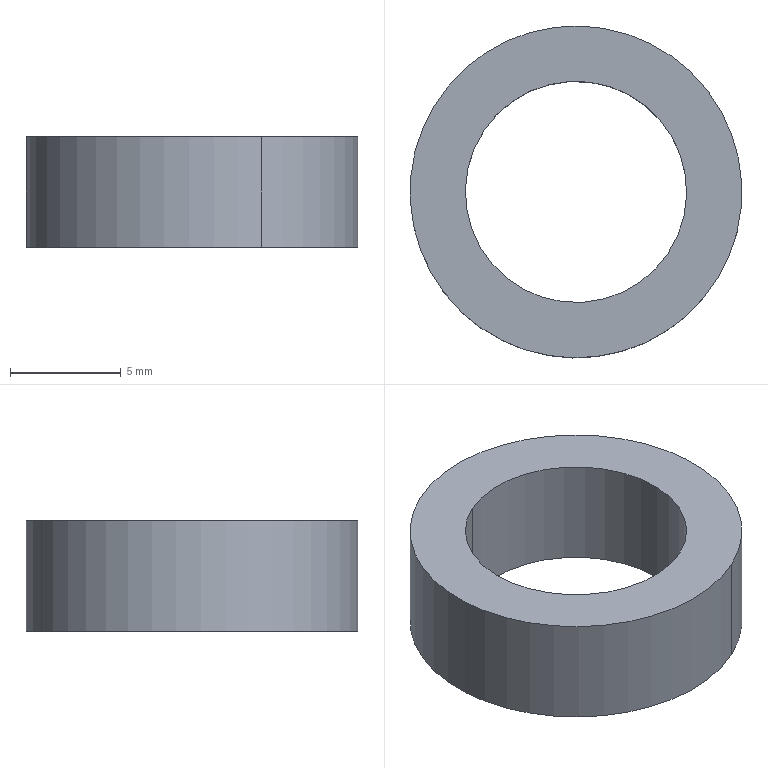Component | SolidWorks | RetainingRing-3 | 1 solid | 6 faces | box 15 x 15 x 5 mm | volume 491 mm3 | cylinder 4 | plane 2 | commonest cylinder face diameters 10 x2 15 x2
build123d program:
from build123d import *

# Parameters (mm, degrees)
SKETCH1_R           = 7.5
SKETCH1_R_2         = 5
BOSS_EXTRUDE1_DEPTH = 5


with BuildPart() as part:
    # Sketch1 → Boss-Extrude1 (new body)
    with BuildSketch(Plane.XY):
        with Locations((215.746, 95.507)):
            Circle(SKETCH1_R)
        with Locations((215.746, 95.507)):
            Circle(SKETCH1_R_2, mode=Mode.SUBTRACT)
    extrude(amount=BOSS_EXTRUDE1_DEPTH)


solid = part.part

# Placed as in the assembly
solid = solid.moved(Location((-435.956, -47.976, -42.818), (0, 0, 0)))
STEP:
#1=COLOUR_RGB('',0.7922,0.8196,0.9333);
#2=FILL_AREA_STYLE_COLOUR('',#1);
#3=FILL_AREA_STYLE('',(#2));
#4=SURFACE_STYLE_FILL_AREA(#3);
#5=SURFACE_SIDE_STYLE('',(#4));
#6=SURFACE_STYLE_USAGE(.BOTH.,#5);
#7=PRESENTATION_STYLE_ASSIGNMENT((#6));
#8=CARTESIAN_POINT('',(-8.752,2.05,-1.686));
#9=VERTEX_POINT('',#8);
#10=CARTESIAN_POINT('',(-8.588,1.692,-1.686));
#11=VERTEX_POINT('',#10);
#12=CARTESIAN_POINT('',(-8.67,1.871,-1.686));
#13=DIRECTION('',(0.,-0.,-1.));
#14=DIRECTION('',(0.4168,-0.909,0.));
#15=AXIS2_PLACEMENT_3D('',#12,#13,#14);
#16=CIRCLE('',#15,0.1969);
#17=EDGE_CURVE('',#9,#11,#16,.T.);
#18=ORIENTED_EDGE('',*,*,#17,.T.);
#19=CARTESIAN_POINT('',(-8.588,1.692,-1.489));
#20=VERTEX_POINT('',#19);
#21=CARTESIAN_POINT('',(-8.588,1.692,-1.686));
#22=DIRECTION('',(-0.,0.,1.));
#23=VECTOR('',#22,39.37);
#24=LINE('',#21,#23);
#25=EDGE_CURVE('',#11,#20,#24,.T.);
#26=ORIENTED_EDGE('',*,*,#25,.T.);
#27=CARTESIAN_POINT('',(-8.752,2.05,-1.489));
#28=VERTEX_POINT('',#27);
#29=CARTESIAN_POINT('',(-8.67,1.871,-1.489));
#30=DIRECTION('',(0.,-0.,-1.));
#31=DIRECTION('',(0.4168,-0.909,0.));
#32=AXIS2_PLACEMENT_3D('',#29,#30,#31);
#33=CIRCLE('',#32,0.1969);
#34=EDGE_CURVE('',#28,#20,#33,.T.);
#35=ORIENTED_EDGE('',*,*,#34,.F.);
#36=CARTESIAN_POINT('',(-8.752,2.05,-1.686));
#37=DIRECTION('',(-0.,0.,1.));
#38=VECTOR('',#37,39.37);
#39=LINE('',#36,#38);
#40=EDGE_CURVE('',#9,#28,#39,.T.);
#41=ORIENTED_EDGE('',*,*,#40,.F.);
#42=EDGE_LOOP('',(#18,#26,#35,#41));
#43=FACE_OUTER_BOUND('',#42,.T.);
#44=CARTESIAN_POINT('',(-8.67,1.871,-1.686));
#45=DIRECTION('',(-0.,0.,1.));
#46=DIRECTION('',(-0.4168,0.909,0.));
#47=AXIS2_PLACEMENT_3D('',#44,#45,#46);
#48=CYLINDRICAL_SURFACE('',#47,0.1969);
#49=ADVANCED_FACE('',(#43),#48,.F.);
#50=CARTESIAN_POINT('',(-8.547,1.603,-1.686));
#51=VERTEX_POINT('',#50);
#52=CARTESIAN_POINT('',(-8.793,2.14,-1.686));
#53=VERTEX_POINT('',#52);
#54=CARTESIAN_POINT('',(-8.67,1.871,-1.686));
#55=DIRECTION('',(0.,-0.,-1.));
#56=DIRECTION('',(0.4168,-0.909,0.));
#57=AXIS2_PLACEMENT_3D('',#54,#55,#56);
#58=CIRCLE('',#57,0.2953);
#59=EDGE_CURVE('',#51,#53,#58,.T.);
#60=ORIENTED_EDGE('',*,*,#59,.F.);
#61=CARTESIAN_POINT('',(-8.547,1.603,-1.489));
#62=VERTEX_POINT('',#61);
#63=CARTESIAN_POINT('',(-8.547,1.603,-1.686));
#64=DIRECTION('',(-0.,0.,1.));
#65=VECTOR('',#64,39.37);
#66=LINE('',#63,#65);
#67=EDGE_CURVE('',#51,#62,#66,.T.);
#68=ORIENTED_EDGE('',*,*,#67,.T.);
#69=CARTESIAN_POINT('',(-8.793,2.14,-1.489));
#70=VERTEX_POINT('',#69);
#71=CARTESIAN_POINT('',(-8.67,1.871,-1.489));
#72=DIRECTION('',(0.,-0.,-1.));
#73=DIRECTION('',(0.4168,-0.909,0.));
#74=AXIS2_PLACEMENT_3D('',#71,#72,#73);
#75=CIRCLE('',#74,0.2953);
#76=EDGE_CURVE('',#62,#70,#75,.T.);
#77=ORIENTED_EDGE('',*,*,#76,.T.);
#78=CARTESIAN_POINT('',(-8.793,2.14,-1.686));
#79=DIRECTION('',(-0.,0.,1.));
#80=VECTOR('',#79,39.37);
#81=LINE('',#78,#80);
#82=EDGE_CURVE('',#53,#70,#81,.T.);
#83=ORIENTED_EDGE('',*,*,#82,.F.);
#84=EDGE_LOOP('',(#60,#68,#77,#83));
#85=FACE_OUTER_BOUND('',#84,.T.);
#86=CARTESIAN_POINT('',(-8.67,1.871,-1.686));
#87=DIRECTION('',(-0.,0.,1.));
#88=DIRECTION('',(-0.4168,0.909,0.));
#89=AXIS2_PLACEMENT_3D('',#86,#87,#88);
#90=CYLINDRICAL_SURFACE('',#89,0.2953);
#91=ADVANCED_FACE('',(#85),#90,.T.);
#92=CARTESIAN_POINT('',(-8.67,1.871,-1.686));
#93=DIRECTION('',(0.,-0.,-1.));
#94=DIRECTION('',(0.4168,-0.909,0.));
#95=AXIS2_PLACEMENT_3D('',#92,#93,#94);
#96=CIRCLE('',#95,0.2953);
#97=EDGE_CURVE('',#53,#51,#96,.T.);
#98=ORIENTED_EDGE('',*,*,#97,.T.);
#99=ORIENTED_EDGE('',*,*,#59,.T.);
#100=EDGE_LOOP('',(#98,#99));
#101=FACE_OUTER_BOUND('',#100,.T.);
#102=ORIENTED_EDGE('',*,*,#17,.F.);
#103=CARTESIAN_POINT('',(-8.67,1.871,-1.686));
#104=DIRECTION('',(0.,-0.,-1.));
#105=DIRECTION('',(0.4168,-0.909,0.));
#106=AXIS2_PLACEMENT_3D('',#103,#104,#105);
#107=CIRCLE('',#106,0.1969);
#108=EDGE_CURVE('',#11,#9,#107,.T.);
#109=ORIENTED_EDGE('',*,*,#108,.F.);
#110=EDGE_LOOP('',(#102,#109));
#111=FACE_BOUND('',#110,.T.);
#112=CARTESIAN_POINT('',(-8.67,1.871,-1.686));
#113=DIRECTION('',(0.,-0.,-1.));
#114=DIRECTION('',(0.4168,-0.909,0.));
#115=AXIS2_PLACEMENT_3D('',#112,#113,#114);
#116=PLANE('',#115);
#117=ADVANCED_FACE('',(#101,#111),#116,.T.);
#118=CARTESIAN_POINT('',(-8.67,1.871,-1.489));
#119=DIRECTION('',(0.,-0.,-1.));
#120=DIRECTION('',(0.4168,-0.909,0.));
#121=AXIS2_PLACEMENT_3D('',#118,#119,#120);
#122=CIRCLE('',#121,0.2953);
#123=EDGE_CURVE('',#70,#62,#122,.T.);
#124=ORIENTED_EDGE('',*,*,#123,.F.);
#125=ORIENTED_EDGE('',*,*,#76,.F.);
#126=EDGE_LOOP('',(#124,#125));
#127=FACE_OUTER_BOUND('',#126,.T.);
#128=ORIENTED_EDGE('',*,*,#34,.T.);
#129=CARTESIAN_POINT('',(-8.67,1.871,-1.489));
#130=DIRECTION('',(0.,-0.,-1.));
#131=DIRECTION('',(0.4168,-0.909,0.));
#132=AXIS2_PLACEMENT_3D('',#129,#130,#131);
#133=CIRCLE('',#132,0.1969);
#134=EDGE_CURVE('',#20,#28,#133,.T.);
#135=ORIENTED_EDGE('',*,*,#134,.T.);
#136=EDGE_LOOP('',(#128,#135));
#137=FACE_BOUND('',#136,.T.);
#138=CARTESIAN_POINT('',(-8.67,1.871,-1.489));
#139=DIRECTION('',(0.,-0.,-1.));
#140=DIRECTION('',(0.4168,-0.909,0.));
#141=AXIS2_PLACEMENT_3D('',#138,#139,#140);
#142=PLANE('',#141);
#143=ADVANCED_FACE('',(#127,#137),#142,.F.);
#144=ORIENTED_EDGE('',*,*,#67,.F.);
#145=ORIENTED_EDGE('',*,*,#97,.F.);
#146=ORIENTED_EDGE('',*,*,#82,.T.);
#147=ORIENTED_EDGE('',*,*,#123,.T.);
#148=EDGE_LOOP('',(#144,#145,#146,#147));
#149=FACE_OUTER_BOUND('',#148,.T.);
#150=CARTESIAN_POINT('',(-8.67,1.871,-1.686));
#151=DIRECTION('',(-0.,0.,1.));
#152=DIRECTION('',(-0.4168,0.909,0.));
#153=AXIS2_PLACEMENT_3D('',#150,#151,#152);
#154=CYLINDRICAL_SURFACE('',#153,0.2953);
#155=ADVANCED_FACE('',(#149),#154,.T.);
#156=ORIENTED_EDGE('',*,*,#25,.F.);
#157=ORIENTED_EDGE('',*,*,#108,.T.);
#158=ORIENTED_EDGE('',*,*,#40,.T.);
#159=ORIENTED_EDGE('',*,*,#134,.F.);
#160=EDGE_LOOP('',(#156,#157,#158,#159));
#161=FACE_OUTER_BOUND('',#160,.T.);
#162=CARTESIAN_POINT('',(-8.67,1.871,-1.686));
#163=DIRECTION('',(-0.,0.,1.));
#164=DIRECTION('',(-0.4168,0.909,0.));
#165=AXIS2_PLACEMENT_3D('',#162,#163,#164);
#166=CYLINDRICAL_SURFACE('',#165,0.1969);
#167=ADVANCED_FACE('',(#161),#166,.F.);
#168=CLOSED_SHELL('',(#49,#91,#117,#143,#155,#167));
#169=MANIFOLD_SOLID_BREP('',#168);
#170=STYLED_ITEM('',(#7),#169);
#171=PRESENTATION_LAYER_ASSIGNMENT('','',(#170));
#172=(LENGTH_UNIT()NAMED_UNIT(*)SI_UNIT($,.METRE.));
#173=LENGTH_MEASURE_WITH_UNIT(LENGTH_MEASURE(0.0254),#172);
#174=DIMENSIONAL_EXPONENTS(1.,0.,0.,0.,0.,0.,0.);
#175=(CONVERSION_BASED_UNIT('',#173)LENGTH_UNIT()NAMED_UNIT(#174));
#176=UNCERTAINTY_MEASURE_WITH_UNIT(LENGTH_MEASURE(0.00001),#175,'','');
#177=(NAMED_UNIT(*)PLANE_ANGLE_UNIT()SI_UNIT($,.RADIAN.));
#178=(NAMED_UNIT(*)SI_UNIT($,.STERADIAN.)SOLID_ANGLE_UNIT());
#179=(GEOMETRIC_REPRESENTATION_CONTEXT(3)GLOBAL_UNCERTAINTY_ASSIGNED_CONTEXT((#176))GLOBAL_UNIT_ASSIGNED_CONTEXT((#175,#177,#178))REPRESENTATION_CONTEXT('',''));
#180=MECHANICAL_DESIGN_GEOMETRIC_PRESENTATION_REPRESENTATION('',(#170),#179);
#181=CARTESIAN_POINT('',(0.,0.,0.));
#182=DIRECTION('',(0.,0.,1.));
#183=DIRECTION('',(1.,0.,0.));
#184=AXIS2_PLACEMENT_3D('',#181,#182,#183);
#185=(LENGTH_UNIT()NAMED_UNIT(*)SI_UNIT($,.METRE.));
#186=LENGTH_MEASURE_WITH_UNIT(LENGTH_MEASURE(0.0254),#185);
#187=DIMENSIONAL_EXPONENTS(1.,0.,0.,0.,0.,0.,0.);
#188=(CONVERSION_BASED_UNIT('',#186)LENGTH_UNIT()NAMED_UNIT(#187));
#189=UNCERTAINTY_MEASURE_WITH_UNIT(LENGTH_MEASURE(0.00001),#188,'','');
#190=(NAMED_UNIT(*)PLANE_ANGLE_UNIT()SI_UNIT($,.RADIAN.));
#191=(NAMED_UNIT(*)SI_UNIT($,.STERADIAN.)SOLID_ANGLE_UNIT());
#192=(GEOMETRIC_REPRESENTATION_CONTEXT(3)GLOBAL_UNCERTAINTY_ASSIGNED_CONTEXT((#189))GLOBAL_UNIT_ASSIGNED_CONTEXT((#188,#190,#191))REPRESENTATION_CONTEXT('',''));
#193=ADVANCED_BREP_SHAPE_REPRESENTATION('',(#169,#184),#192);